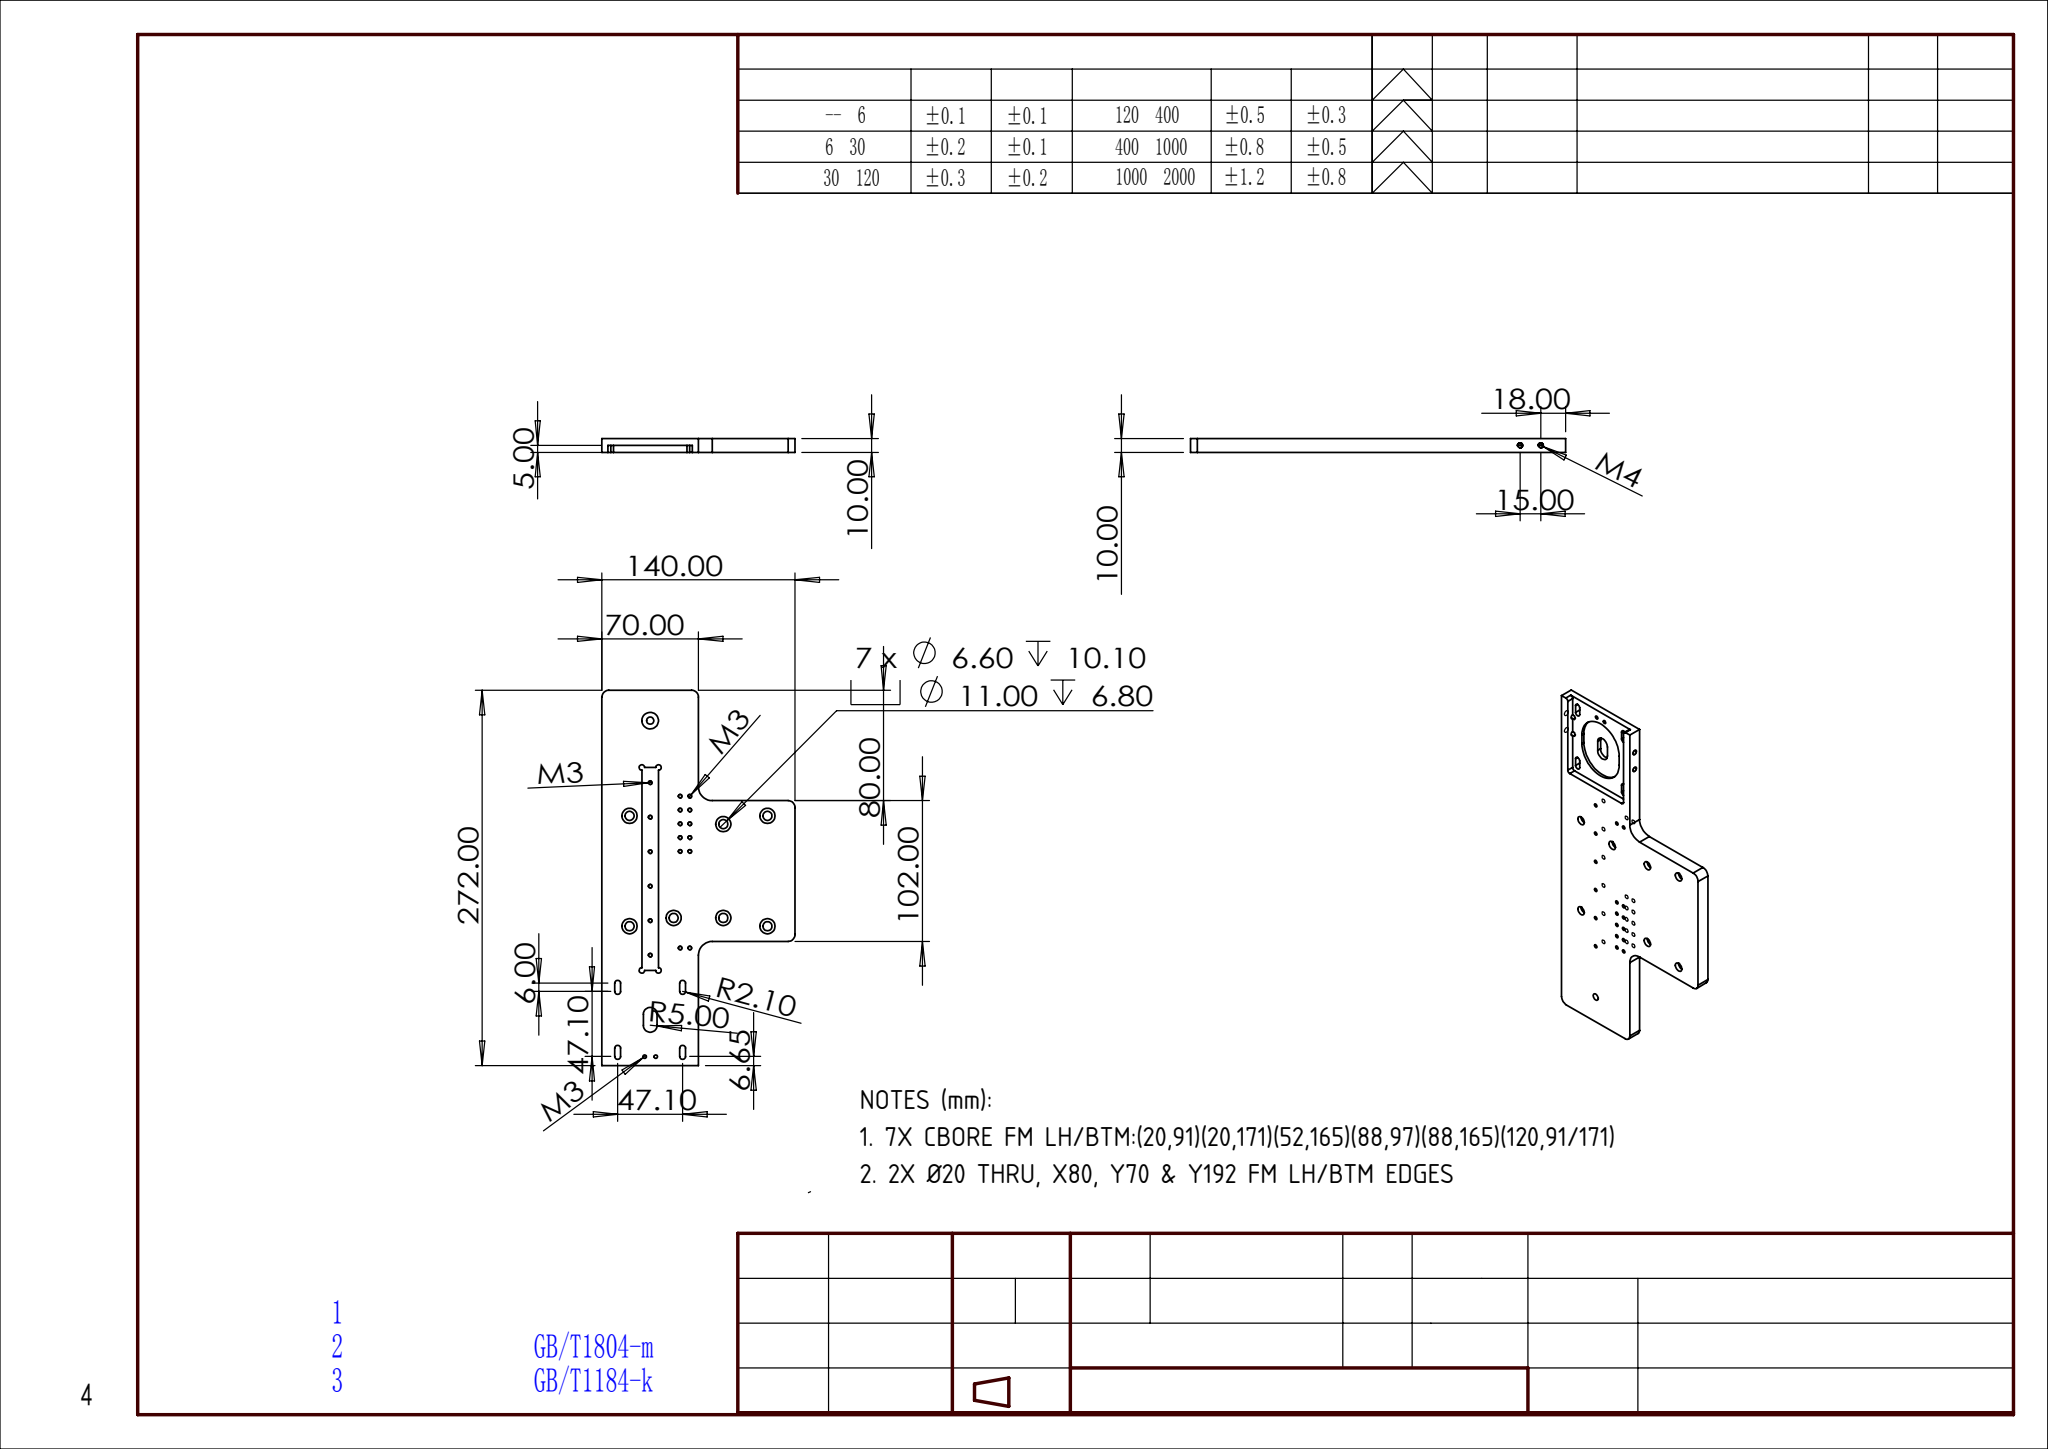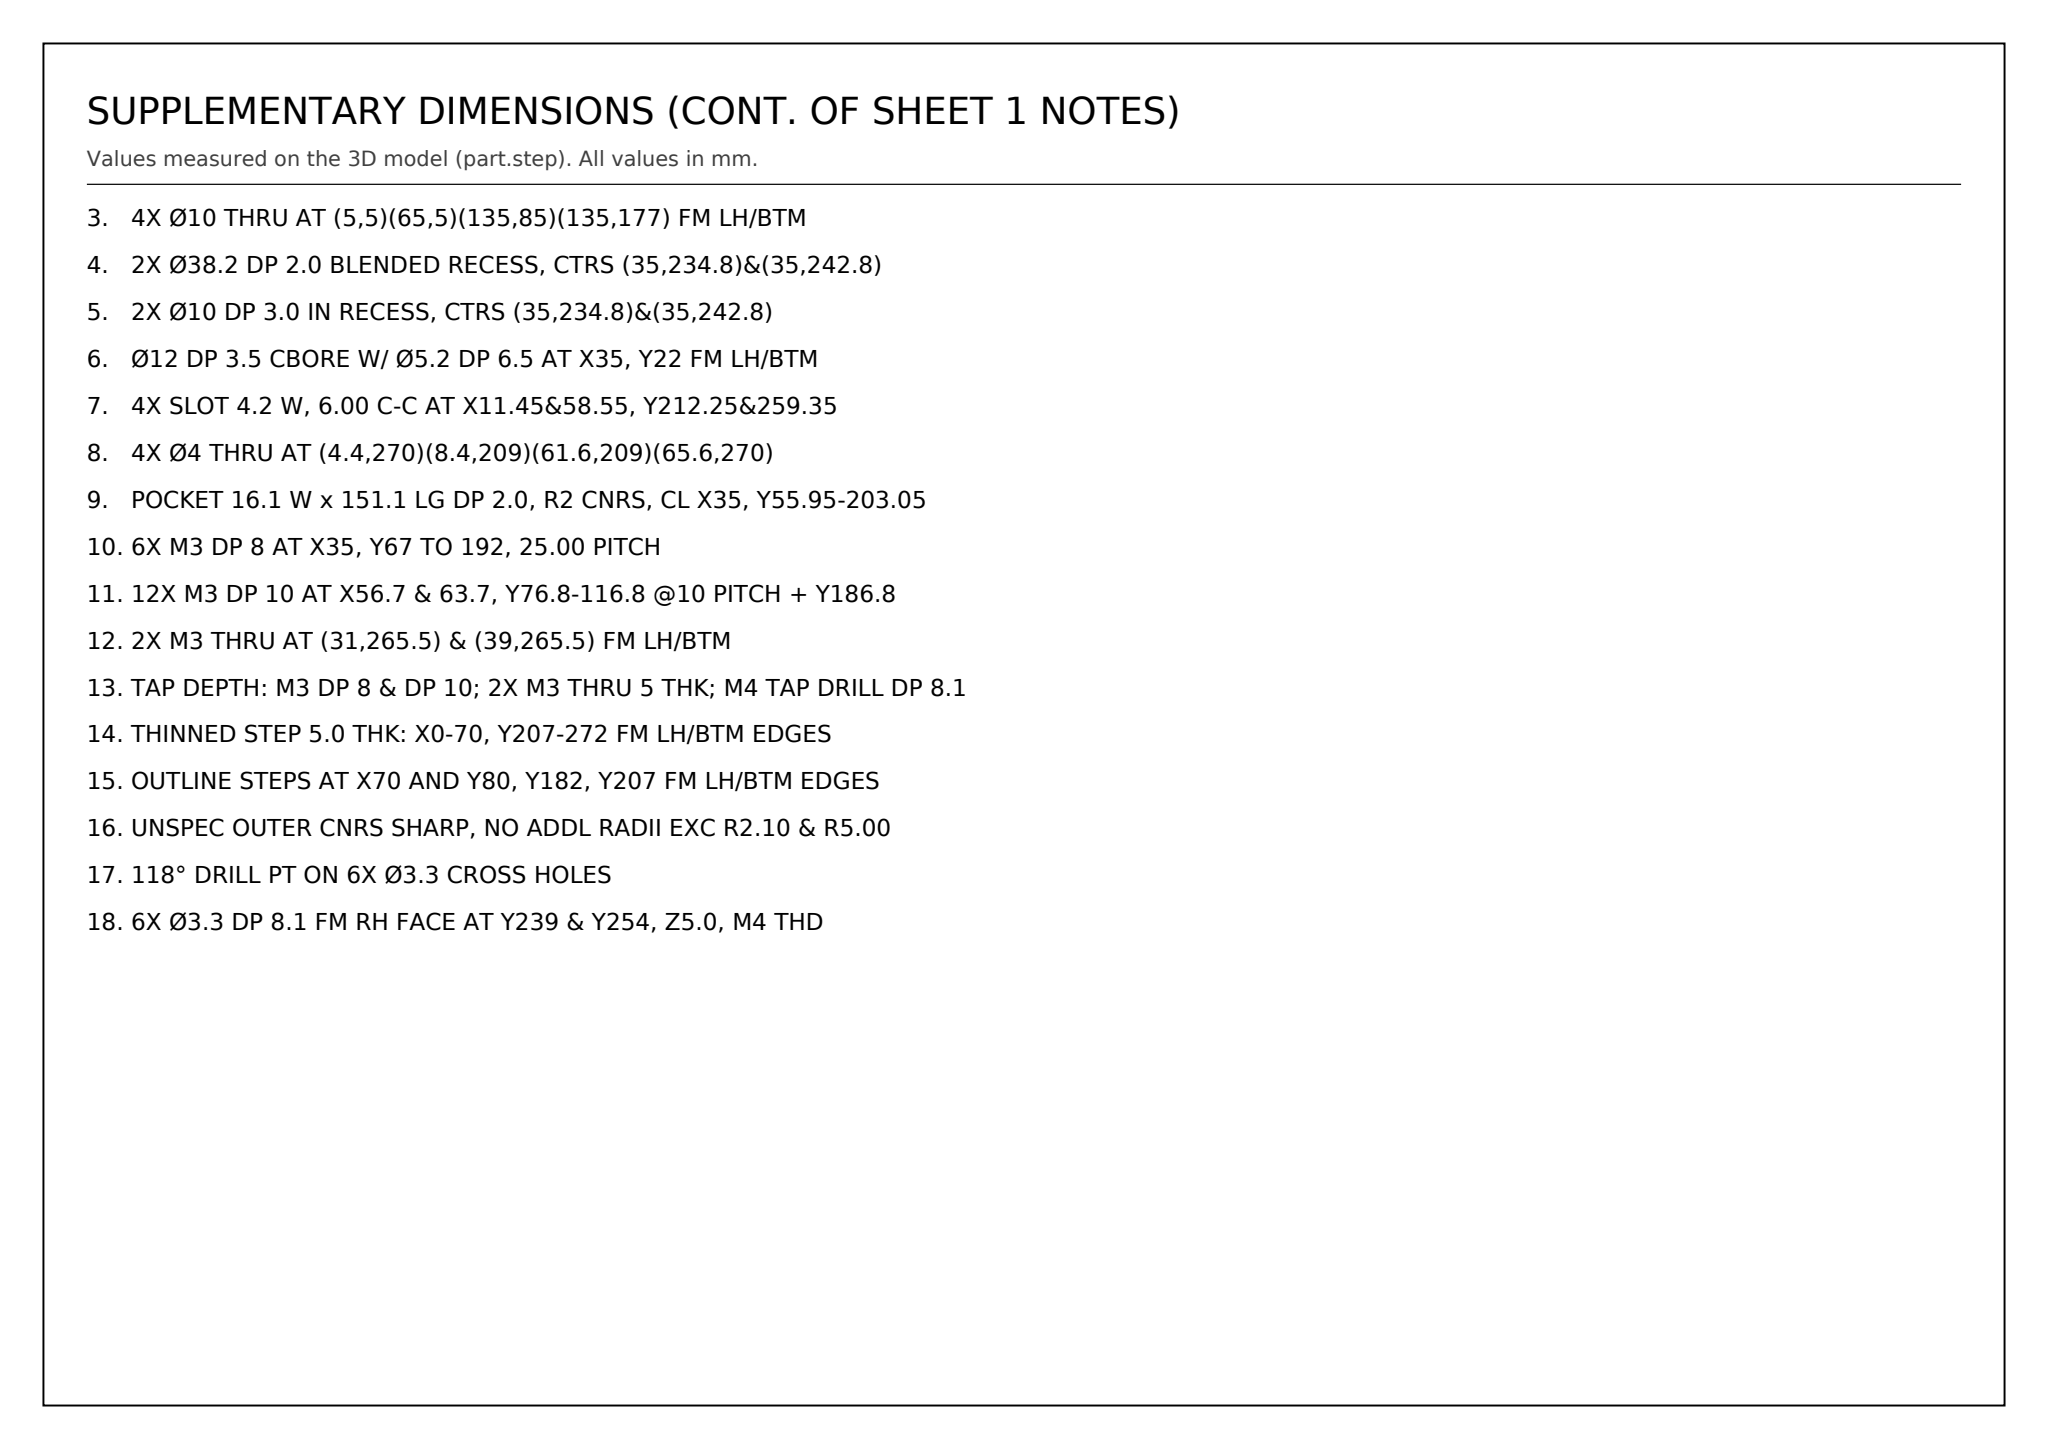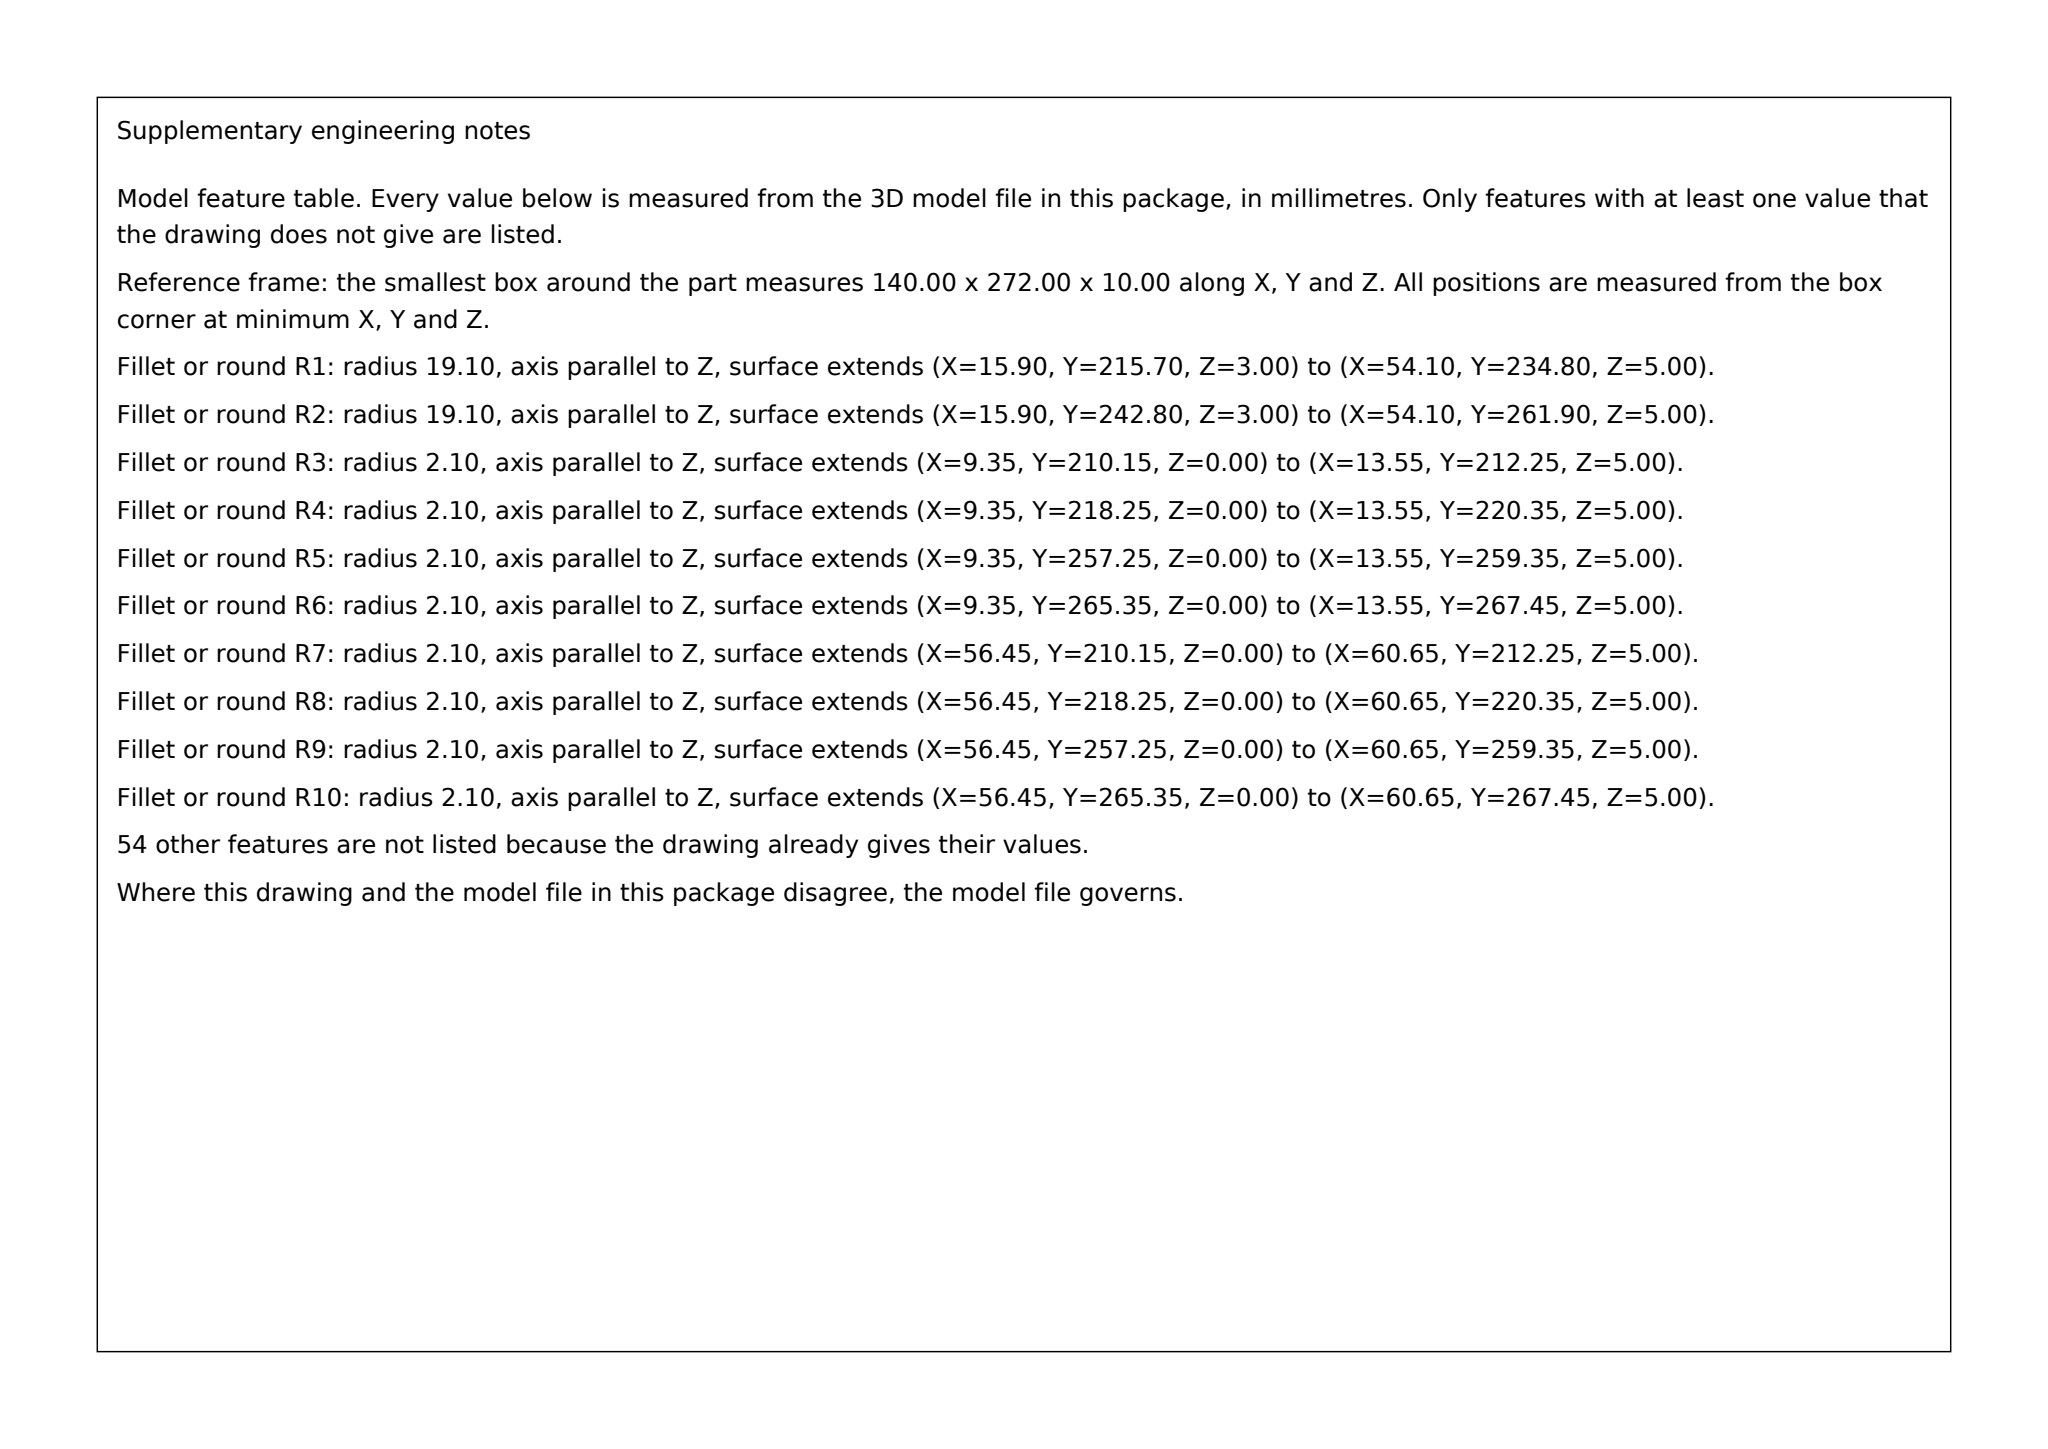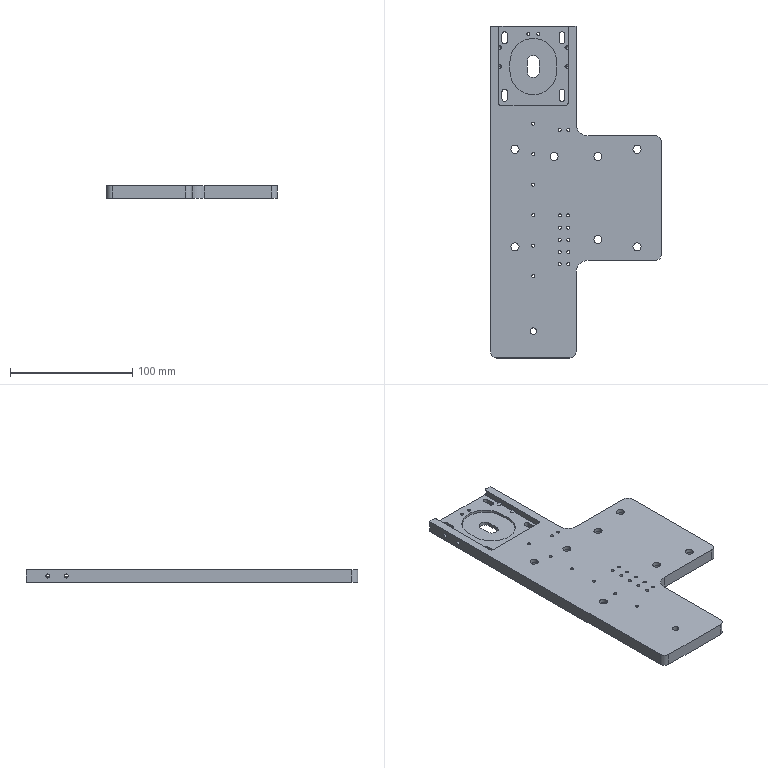Part | SolidWorks | mm | 1 solid | 154 faces | box 140 x 272 x 10 mm | volume 228678 mm3 | cylinder 108 | plane 40 | cone 6 | commonest cylinder face diameters 2.5 x40 11 x14 6.6 x14 4 x10 3.3 x8 4.2 x8 10 x6 5.2 x2
Drawing notes:
7X CBORE FM LH/BTM:(20,91)(20,171)(52,165)(88,97)(88,165)(120,91/171) | from the solid: Ø6.6/Ø11 cyl pairs at (20,91)(20,171)(52,165)(88,97)(88,165)(120,91)(120,171)
2X Ø20 THRU, X80, Y70 & Y192 FM LH/BTM EDGES | from the solid: [20.0,'z',[80,70],10] and [20.0,'z',[80,192],10]; bbox z=10
4X Ø10 THRU AT (5,5)(65,5)(135,85)(135,177) FM LH/BTM | from the solid: [10.0,'z',[5,5],10][65,5][135,85][135,177] length 10 = full thk
2X Ø38.2 DP 2.0 BLENDED RECESS, CTRS (35,234.8)&(35,242.8) | from the solid: [38.2,'z',[35,234.8],2.0] and [38.2,'z',[35,242.8],2.0]
2X Ø10 DP 3.0 IN RECESS, CTRS (35,234.8)&(35,242.8) | from the solid: [10.0,'z',[35,234.8],3.0] and [10.0,'z',[35,242.8],3.0]
Ø12 DP 3.5 CBORE W/ Ø5.2 DP 6.5 AT X35, Y22 FM LH/BTM | from the solid: [12.0,'z',[35,22],3.5] and [5.2,'z',[35,22],6.5]
4X SLOT 4.2 W, 6.00 C-C AT X11.45&58.55, Y212.25&259.35 | from the solid: 8X Ø4.2 at X11.45/58.55, Y212.25,218.25,259.35,265.35; x planes 9.35/13.55, 56.45/60.65
4X Ø4 THRU AT (4.4,270)(8.4,209)(61.6,209)(65.6,270) | from the solid: [4.0,'z',[4.4,270],5][8.4,209][61.6,209][65.6,270], 5 thk region
POCKET 16.1 W x 151.1 LG DP 2.0, R2 CNRS, CL X35, Y55.95-203.05 | from the solid: Ø4 ↧2.0 ends at (28.95/41.05, 55.95/203.05); x planes 28.95,41.05; y planes 55.95,203.05
6X M3 DP 8 AT X35, Y67 TO 192, 25.00 PITCH | from the solid: Ø2.5 z-holes at X35, Y67,92,117,142,167,192, length 8
12X M3 DP 10 AT X56.7 & 63.7, Y76.8-116.8 @10 PITCH + Y186.8 | from the solid: Ø2.5 len 10 at X56.7/63.7, Y76.8,86.8,96.8,106.8,116.8,186.8
2X M3 THRU AT (31,265.5) & (39,265.5) FM LH/BTM | from the solid: Ø2.5 len 5 at (31,265.5)(39,265.5) in 5 thk region
TAP DEPTH: M3 DP 8 & DP 10; 2X M3 THRU 5 THK; M4 TAP DRILL DP 8.1 | from the solid: Ø2.5 lengths 8, 10, 5; Ø3.3 x-axis length 8.1
THINNED STEP 5.0 THK: X0-70, Y207-272 FM LH/BTM EDGES | from the solid: z plane 5.0; x plane 70; y plane 207; holes at Y209-270 only 5 deep thru
OUTLINE STEPS AT X70 AND Y80, Y182, Y207 FM LH/BTM EDGES | from the solid: axis planes x=70 (2), y=80, y=182, y=207
UNSPEC OUTER CNRS SHARP, NO ADDL RADII EXC R2.10 & R5.00 | from the solid: fillet_radii list empty
118° DRILL PT ON 6X Ø3.3 CROSS HOLES | from the solid: cones [118.0, 3.3, 6]
6X Ø3.3 DP 8.1 FM RH FACE AT Y239 & Y254, Z5.0, M4 THD | from the solid: [3.3,'x',[null,239,5],8.1] and [3.3,'x',[null,254,5],8.1]
build123d program:
from build123d import *

# Parameters (mm, degrees)
SKETCH1_W                                            = 70
SKETCH1_H                                            = 272
BOSS_EXTRUDE1_DEPTH                                  = 10
SKETCH2_W                                            = 57.2
SKETCH2_H                                            = 65
CUT_EXTRUDE1_DEPTH                                   = 5
CUT_EXTRUDE2_DEPTH                                   = 10
CUT_EXTRUDE3_DEPTH                                   = 2
SKETCH7_W                                            = 12.1
SKETCH7_H                                            = 147.1
CUT_EXTRUDE4_DEPTH                                   = 2
M3_TAPPED_HOLE1_D                                    = 2.5
CUT_EXTRUDE12_DEPTH                                  = 141.606
SKETCH10_R                                           = 6
CUT_EXTRUDE5_DEPTH                                   = 3.5
F_5_2_5_2_DIAMETER_HOLE1_D                           = 5.2
SKETCH32_R                                           = 2
CUT_EXTRUDE11_DEPTH                                  = 2
M3_TAPPED_HOLE2_D                                    = 2.5
M3_TAPPED_HOLE2_DEPTH                                = 11.5
M3_TAPPED_HOLE2_TIP                                  = 0.7511
M4_TAPPED_HOLE7_AT_2_COUNT                           = 2
M4_TAPPED_HOLE7_AT_2_PITCH                           = 15
SKETCH64_W                                           = 70
SKETCH64_H                                           = 102
BOSS_EXTRUDE2_DEPTH                                  = 10
HOLE_SIZE_ACCORDING_TO_TYPE_OF_HEXAGON_S_D           = 6.6
HOLE_SIZE_ACCORDING_TO_TYPE_OF_HEXAGON_S_DEPTH       = 10.1
HOLE_SIZE_ACCORDING_TO_TYPE_OF_HEXAGON_S_CBORE_D     = 11
HOLE_SIZE_ACCORDING_TO_TYPE_OF_HEXAGON_S_CBORE_DEPTH = 6.8
HOLE_SIZE_ACCORDING_TO_TYPE_OF_HEXAGON_S_TIP         = 1.983
FILLET3_R                                            = 10
FILLET2_R                                            = 5
FILLET4_R                                            = 2


with BuildPart() as part:
    # Sketch1 → Boss-Extrude1 (new body)
    with BuildSketch(Plane.XY):
        Rectangle(SKETCH1_W, SKETCH1_H)
    extrude(amount=BOSS_EXTRUDE1_DEPTH)

    # Sketch2 → Cut-Extrude1 (cut)
    with BuildSketch(Plane.XY.offset(10)):
        with Locations((0, 103.5)):
            Rectangle(SKETCH2_W, SKETCH2_H)
    extrude(amount=-CUT_EXTRUDE1_DEPTH, mode=Mode.SUBTRACT)

    # Sketch4 → Cut-Extrude2 (cut)
    with BuildSketch(Plane.XY.offset(10)):
        with BuildLine():
            Line((25.65, 129.35), (25.65, 123.35))
            ThreePointArc((25.65, 123.35), (23.55, 121.25), (21.45, 123.35))
            Line((21.45, 123.35), (21.45, 129.35))
            ThreePointArc((21.45, 129.35), (23.55, 131.45), (25.65, 129.35))
        make_face()
        with BuildLine():
            Line((-25.65, 123.35), (-25.65, 129.35))
            ThreePointArc((-25.65, 129.35), (-23.55, 131.45), (-21.45, 129.35))
            Line((-21.45, 129.35), (-21.45, 123.35))
            ThreePointArc((-21.45, 123.35), (-23.55, 121.25), (-25.65, 123.35))
        make_face()
        with BuildLine():
            Line((-25.65, 76.25), (-25.65, 82.25))
            ThreePointArc((-25.65, 82.25), (-23.55, 84.35), (-21.45, 82.25))
            Line((-21.45, 82.25), (-21.45, 76.25))
            ThreePointArc((-21.45, 76.25), (-23.55, 74.15), (-25.65, 76.25))
        make_face()
        with BuildLine():
            Line((21.45, 76.25), (21.45, 82.25))
            ThreePointArc((21.45, 82.25), (23.55, 84.35), (25.65, 82.25))
            Line((25.65, 82.25), (25.65, 76.25))
            ThreePointArc((25.65, 76.25), (23.55, 74.15), (21.45, 76.25))
        make_face()
    extrude(amount=-CUT_EXTRUDE2_DEPTH, mode=Mode.SUBTRACT)

    # Sketch5 → Cut-Extrude3 (cut)
    with BuildSketch(Plane(origin=(0, 0, 5), x_dir=(-1, 0, 0), z_dir=(0, 0, -1))):
        with BuildLine():
            Line((-19.1, 98.8), (-19.1, 106.8))
            ThreePointArc((-19.1, 106.8), (0, 125.9), (19.1, 106.8))
            Line((19.1, 106.8), (19.1, 98.8))
            ThreePointArc((19.1, 98.8), (0, 79.7), (-19.1, 98.8))
        make_face()
    extrude(amount=CUT_EXTRUDE3_DEPTH, mode=Mode.SUBTRACT)

    # Sketch7 → Cut-Extrude4 (cut)
    with BuildSketch(Plane(origin=(0, 0, 0), x_dir=(-1, 0, 0), z_dir=(0, 0, -1))):
        with Locations((0, -6.5)):
            Rectangle(SKETCH7_W, SKETCH7_H)
    extrude(amount=-CUT_EXTRUDE4_DEPTH, mode=Mode.SUBTRACT)

    # M3 Tapped Hole1 (through all)
    with Locations(Plane(origin=(0, 0, 0), x_dir=(-1, 0, 0), z_dir=(0, 0, -1))):
        with Locations((-28.7, 50.8), (-21.7, 50.8), (-28.7, -59.2), (-21.7, -59.2), (-28.7, -49.2), (-21.7, -49.2), (-28.7, -39.2), (-21.7, -39.2), (-28.7, -29.2), (-21.7, -29.2), (-28.7, -19.2), (-21.7, -19.2), (4, 129.5), (-4, 129.5)):
            Hole(M3_TAPPED_HOLE1_D / 2)

    # Sketch33 → Cut-Extrude12 (cut, through all)
    with BuildSketch(Plane.XY.offset(3)):
        with BuildLine():
            Line((-5, 98.8), (-5, 106.8))
            ThreePointArc((-5, 106.8), (0, 111.8), (5, 106.8))
            Line((5, 106.8), (5, 98.8))
            ThreePointArc((5, 98.8), (0, 93.8), (-5, 98.8))
        make_face()
    extrude(amount=-CUT_EXTRUDE12_DEPTH, mode=Mode.SUBTRACT)

    # Sketch10 → Cut-Extrude5 (cut)
    with BuildSketch(Plane(origin=(0, 0, 0), x_dir=(-1, 0, 0), z_dir=(0, 0, -1))):
        with Locations((0, -114)):
            Circle(SKETCH10_R)
    extrude(amount=-CUT_EXTRUDE5_DEPTH, mode=Mode.SUBTRACT)

    # 5.2 _5.2_ Diameter Hole1 (through all)
    with Locations(Plane(origin=(0, 0, 10), x_dir=(-1, 0, 0), z_dir=(0, 0, 1))):
        with Locations((0, 114)):
            Hole(F_5_2_5_2_DIAMETER_HOLE1_D / 2)

    # Sketch32 → Cut-Extrude11 (cut)
    with BuildSketch(Plane(origin=(0, 0, 0), x_dir=(-1, 0, 0), z_dir=(0, 0, -1))):
        with Locations((6.05, 67.05)):
            Circle(SKETCH32_R)
        with Locations((-6.05, 67.05)):
            Circle(SKETCH32_R)
        with Locations((6.05, -80.05)):
            Circle(SKETCH32_R)
        with Locations((-6.05, -80.05)):
            Circle(SKETCH32_R)
    extrude(amount=-CUT_EXTRUDE11_DEPTH, mode=Mode.SUBTRACT)

    # M3 Tapped Hole2
    with Locations(Plane(origin=(0, 0, 0), x_dir=(-1, 0, 0), z_dir=(0, 0, -1))):
        with Locations((0, 6), (0, -19), (0, -44), (0, -69), (0, 56), (0, 31)):
            Hole(M3_TAPPED_HOLE2_D / 2, depth=M3_TAPPED_HOLE2_DEPTH)
            with Locations((0, 0, -(M3_TAPPED_HOLE2_DEPTH + M3_TAPPED_HOLE2_TIP / 2))):  # 118° drill point
                Cone(0, M3_TAPPED_HOLE2_D / 2, M3_TAPPED_HOLE2_TIP, mode=Mode.SUBTRACT)

    # Sketch60 → M4 Tapped Hole7 (revolve, cut)
    with BuildSketch(Plane(origin=(-35, 103, 5), x_dir=(0, 0, 1), z_dir=(0, 1, 0))):
        Polygon((0, 0), (0, 9.091), (1.65, 8.1), (1.65, 0), align=None)
    m4_tapped_hole7 = revolve(axis=Axis((-41.35, 103, 5), (1, 0, 0)), mode=Mode.SUBTRACT)

    # M4 Tapped Hole7 at 2: M4 Tapped Hole7 ×2
    with Locations(*[(0, i * M4_TAPPED_HOLE7_AT_2_PITCH, 0) for i in range(1, M4_TAPPED_HOLE7_AT_2_COUNT)]):
        add(m4_tapped_hole7, mode=Mode.SUBTRACT)

    # Sketch64 → Boss-Extrude2 (add)
    with BuildSketch(Plane(origin=(0, 0, 0), x_dir=(-1, 0, 0), z_dir=(0, 0, -1))):
        with Locations((-70, -5)):
            Rectangle(SKETCH64_W, SKETCH64_H)
    extrude(amount=-BOSS_EXTRUDE2_DEPTH)

    # Hole Size_According to_Type of Hexagon S
    with Locations(Plane(origin=(0, 0, 0), x_dir=(-1, 0, 0), z_dir=(0, 0, -1))):
        with Locations((-85, 35), (-53, 29), (-17, 29), (15, 35), (-85, -45), (-53, -39), (15, -45)):
            CounterBoreHole(HOLE_SIZE_ACCORDING_TO_TYPE_OF_HEXAGON_S_D / 2, HOLE_SIZE_ACCORDING_TO_TYPE_OF_HEXAGON_S_CBORE_D / 2, HOLE_SIZE_ACCORDING_TO_TYPE_OF_HEXAGON_S_CBORE_DEPTH, depth=HOLE_SIZE_ACCORDING_TO_TYPE_OF_HEXAGON_S_DEPTH)
            with Locations((0, 0, -(HOLE_SIZE_ACCORDING_TO_TYPE_OF_HEXAGON_S_DEPTH + HOLE_SIZE_ACCORDING_TO_TYPE_OF_HEXAGON_S_TIP / 2))):  # 118° drill point
                Cone(0, HOLE_SIZE_ACCORDING_TO_TYPE_OF_HEXAGON_S_D / 2, HOLE_SIZE_ACCORDING_TO_TYPE_OF_HEXAGON_S_TIP, mode=Mode.SUBTRACT)

    # Fillet3
    fillet3_edges = [part.edges().sort_by_distance(p)[0] for p in [
        (35, 46, 5),
        (35, -56, 5),
    ]]
    fillet(fillet3_edges, radius=FILLET3_R)

    # Fillet2
    fillet2_edges = [part.edges().sort_by_distance(p)[0] for p in [
        (105, -56, 5),
        (105, 46, 5),
        (35, -136, 5),
        (-35, -136, 5),
    ]]
    fillet(fillet2_edges, radius=FILLET2_R)

    # Fillet4
    fillet4_edges = [part.edges().sort_by_distance(p)[0] for p in [
        (28.6, 136, 7.5),
        (28.6, 71, 7.5),
        (-28.6, 71, 7.5),
        (-28.6, 136, 7.5),
    ]]
    fillet(fillet4_edges, radius=FILLET4_R)

    # Mirror1: M4 Tapped Hole7 across plane
    add(m4_tapped_hole7.mirror(Plane(origin=(0, 0, 0), x_dir=(0, 0, 1), z_dir=(1, 0, 0))), mode=Mode.SUBTRACT)

    # Mirror1 copy 1 sketch → Mirror1 copy 1 (revolve, cut)
    with BuildSketch(Plane(origin=(35, 118, 5), x_dir=(0, 0, 1), z_dir=(0, 1, 0))):
        Polygon((0, 0), (0, -9.091), (1.65, -8.1), (1.65, 0), align=None)
    revolve(axis=Axis((41.35, 118, 5), (1, 0, 0)), mode=Mode.SUBTRACT)


solid = part.part